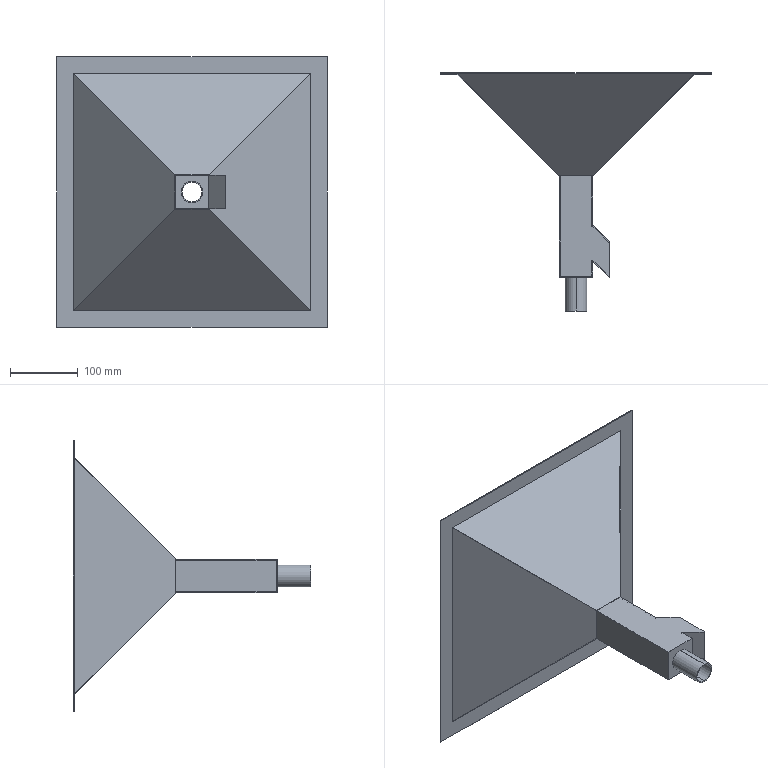Component | SolidWorks | Funnel-1 | 1 solid | 41 faces | volume 369885 mm3 | plane 37 | cylinder 4 | commonest cylinder face diameters 29 x2 32 x2